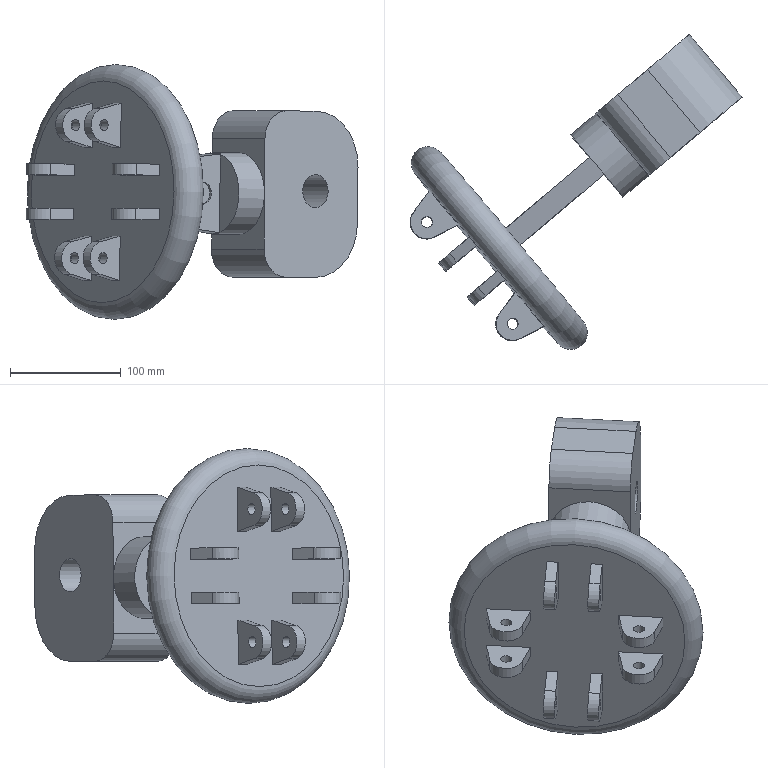Component | NX | BASEPINZAS | 8 solids | 85 faces | volume 2565018 mm3 | plane 58 | cylinder 26 | torus 1 | commonest cylinder face diameters 30 x9 10 x8 20 x4 50 x2 100 x2 73.763 x1